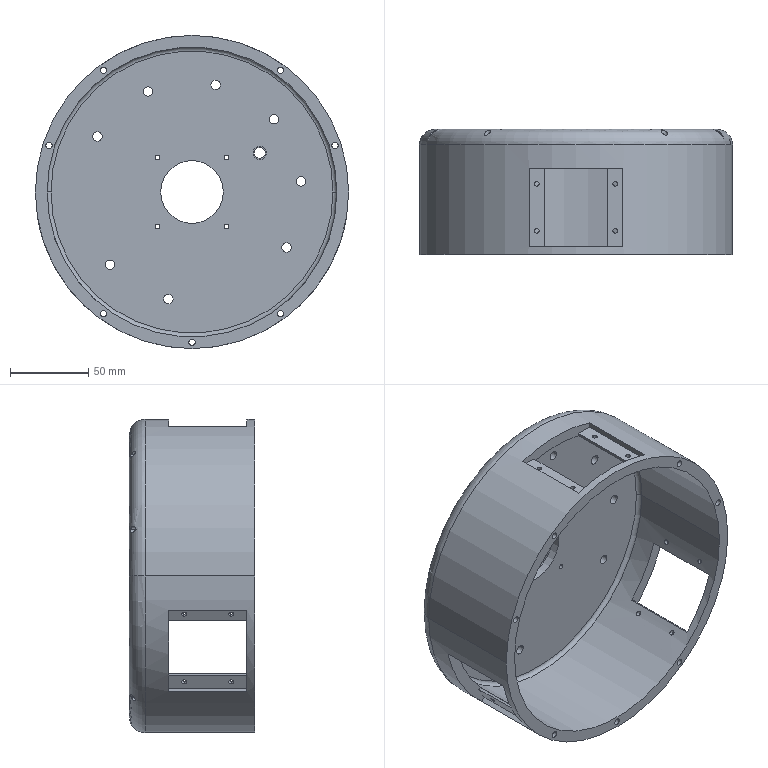Component | SolidWorks | UpperHousing-1 | 1 solid | 106 faces | box 200 x 80 x 200 mm | volume 473499 mm3 | cylinder 72 | plane 28 | torus 6 | commonest cylinder face diameters 3 x32 6 x16 4 x14 8.5 x2 40 x2 185 x2 200 x2 7 x2
build123d program:
from build123d import *

# Parameters (mm, degrees)
SKETCH2_R               = 100
BOSS_EXTRUDE1_DEPTH     = 80
FILLET1_R               = 10
SHELL1_T                = -7.5
CUT_EXTRUDE1_2_REACH    = 164.481
SKETCH3_R               = 2
SKETCH5_W               = 50
SKETCH5_H               = 18.217
CUT_EXTRUDE3_DEPTH      = 20
CIRPATTERN1_COUNT       = 3
SKETCH8_W               = 60
SKETCH8_H               = 50
CUT_EXTRUDE4_DEPTH      = 8
CIRPATTERN2_COUNT       = 3
CUT_EXTRUDE5_REACH      = 232.79
CUT_EXTRUDE5_END_RADIUS = 92.5
SKETCH9_R               = 1.5
CIRPATTERN3_COUNT       = 3
CUT_EXTRUDE6_REACH      = 164.481
SKETCH10_R              = 20
FILLET2_R               = 2
CUT_EXTRUDE7_REACH      = 164.481
SKETCH12_R              = 1.5
CUT_EXTRUDE9_REACH      = 164.481
SKETCH13_R              = 3
CUT_EXTRUDE10_REACH     = 164.481
SKETCH14_R              = 3.5
SKETCH1_R               = 4.25
CUT_EXTRUDE1_DEPTH      = 2.6


with BuildPart() as part:
    # Sketch2 → Boss-Extrude1 (new body)
    with BuildSketch(Plane.XY):
        Circle(SKETCH2_R)
    extrude(amount=BOSS_EXTRUDE1_DEPTH)

    # Fillet1
    fillet1_edges = [part.edges().sort_by_distance(p)[0] for p in [
        (-100, 0, 80),
    ]]
    fillet(fillet1_edges, radius=FILLET1_R)

    # Shell1
    shell1_openings = [part.faces().sort_by_distance(p)[0] for p in [
        (0, 0, 0),
    ]]
    offset(amount=SHELL1_T, openings=shell1_openings, kind=Kind.INTERSECTION)

    # Sketch3 → Cut-Extrude1_2 (cut, up to next)
    with BuildSketch(Plane(origin=(0, 0, 0), x_dir=(-1, 0, 0), z_dir=(0, 0, -1)), mode=Mode.PRIVATE) as cut_extrude1_2_sk1:
        with Locations((0, 96)):
            Circle(SKETCH3_R)
    cut_extrude1_2_tool1 = extrude(cut_extrude1_2_sk1.sketch, amount=-CUT_EXTRUDE1_2_REACH, mode=Mode.PRIVATE) & part.part
    # Sketch3 → Cut-Extrude1_2 (cut, up to next)
    with BuildSketch(Plane(origin=(0, 0, 0), x_dir=(-1, 0, 0), z_dir=(0, 0, -1)), mode=Mode.PRIVATE) as cut_extrude1_2_sk2:
        with Locations((56.427, 77.666)):
            Circle(SKETCH3_R)
    cut_extrude1_2_tool2 = extrude(cut_extrude1_2_sk2.sketch, amount=-CUT_EXTRUDE1_2_REACH, mode=Mode.PRIVATE) & part.part
    # Sketch3 → Cut-Extrude1_2 (cut, up to next)
    with BuildSketch(Plane(origin=(0, 0, 0), x_dir=(-1, 0, 0), z_dir=(0, 0, -1)), mode=Mode.PRIVATE) as cut_extrude1_2_sk3:
        with Locations((91.301, -29.666)):
            Circle(SKETCH3_R)
    cut_extrude1_2_tool3 = extrude(cut_extrude1_2_sk3.sketch, amount=-CUT_EXTRUDE1_2_REACH, mode=Mode.PRIVATE) & part.part
    # Sketch3 → Cut-Extrude1_2 (cut, up to next)
    with BuildSketch(Plane(origin=(0, 0, 0), x_dir=(-1, 0, 0), z_dir=(0, 0, -1)), mode=Mode.PRIVATE) as cut_extrude1_2_sk4:
        with Locations((56.427, -77.666)):
            Circle(SKETCH3_R)
    cut_extrude1_2_tool4 = extrude(cut_extrude1_2_sk4.sketch, amount=-CUT_EXTRUDE1_2_REACH, mode=Mode.PRIVATE) & part.part
    # Sketch3 → Cut-Extrude1_2 (cut, up to next)
    with BuildSketch(Plane(origin=(0, 0, 0), x_dir=(-1, 0, 0), z_dir=(0, 0, -1)), mode=Mode.PRIVATE) as cut_extrude1_2_sk5:
        with Locations((-56.427, -77.666)):
            Circle(SKETCH3_R)
    cut_extrude1_2_tool5 = extrude(cut_extrude1_2_sk5.sketch, amount=-CUT_EXTRUDE1_2_REACH, mode=Mode.PRIVATE) & part.part
    # Sketch3 → Cut-Extrude1_2 (cut, up to next)
    with BuildSketch(Plane(origin=(0, 0, 0), x_dir=(-1, 0, 0), z_dir=(0, 0, -1)), mode=Mode.PRIVATE) as cut_extrude1_2_sk6:
        with Locations((-91.301, -29.666)):
            Circle(SKETCH3_R)
    cut_extrude1_2_tool6 = extrude(cut_extrude1_2_sk6.sketch, amount=-CUT_EXTRUDE1_2_REACH, mode=Mode.PRIVATE) & part.part
    # Sketch3 → Cut-Extrude1_2 (cut, up to next)
    with BuildSketch(Plane(origin=(0, 0, 0), x_dir=(-1, 0, 0), z_dir=(0, 0, -1)), mode=Mode.PRIVATE) as cut_extrude1_2_sk7:
        with Locations((-56.427, 77.666)):
            Circle(SKETCH3_R)
    cut_extrude1_2_tool7 = extrude(cut_extrude1_2_sk7.sketch, amount=-CUT_EXTRUDE1_2_REACH, mode=Mode.PRIVATE) & part.part
    add(cut_extrude1_2_tool1.solids().sort_by_distance((0, 96, 0))[0], mode=Mode.SUBTRACT)
    add(cut_extrude1_2_tool2.solids().sort_by_distance((-56.427, 77.666, 0))[0], mode=Mode.SUBTRACT)
    add(cut_extrude1_2_tool3.solids().sort_by_distance((-91.301, -29.666, 0))[0], mode=Mode.SUBTRACT)
    add(cut_extrude1_2_tool4.solids().sort_by_distance((-56.427, -77.666, 0))[0], mode=Mode.SUBTRACT)
    add(cut_extrude1_2_tool5.solids().sort_by_distance((56.427, -77.666, 0))[0], mode=Mode.SUBTRACT)
    add(cut_extrude1_2_tool6.solids().sort_by_distance((91.301, -29.666, 0))[0], mode=Mode.SUBTRACT)
    add(cut_extrude1_2_tool7.solids().sort_by_distance((56.427, 77.666, 0))[0], mode=Mode.SUBTRACT)

    # Sketch5 → Cut-Extrude3 (cut, symmetric)
    with BuildSketch(Plane(origin=(0, 0, 0), x_dir=(0, 0, -1), z_dir=(1, 0, 0))):
        with Locations((-30, -96.918)):
            Rectangle(SKETCH5_W, SKETCH5_H)
    cut_extrude3 = extrude(amount=CUT_EXTRUDE3_DEPTH, both=True, mode=Mode.SUBTRACT)

    # CirPattern1: Cut-Extrude3 ×3 about axis
    cirpattern1_axis = Axis((0, 0, 0), (0, 0, 1))
    for i in range(1, CIRPATTERN1_COUNT):
        add(cut_extrude3.rotate(cirpattern1_axis, i * 360 / CIRPATTERN1_COUNT), mode=Mode.SUBTRACT)

    # Sketch8 → Cut-Extrude4 (cut)
    with BuildSketch(Plane(origin=(0, -100, 0), x_dir=(1, 0, 0), z_dir=(0, 1, 0))):
        with Locations((0, -30)):
            Rectangle(SKETCH8_W, SKETCH8_H)
    cut_extrude4 = extrude(amount=CUT_EXTRUDE4_DEPTH, mode=Mode.SUBTRACT)

    # CirPattern2: Cut-Extrude4 ×3 about axis
    cirpattern2_axis = Axis((0, 0, 0), (0, 0, 1))
    for i in range(1, CIRPATTERN2_COUNT):
        add(cut_extrude4.rotate(cirpattern2_axis, i * 360 / CIRPATTERN2_COUNT), mode=Mode.SUBTRACT)

    # Cut-Extrude5: up to this cylinder (the profile starts outside it)
    cut_extrude5_end = Plane(origin=(0, 0, 30), z_dir=(0, 0, -1)) * Cylinder(CUT_EXTRUDE5_END_RADIUS, 681.58, mode=Mode.PRIVATE)
    # Sketch9 → Cut-Extrude5 (cut, up to the surface)
    with BuildSketch(Plane.XZ.offset(92), mode=Mode.PRIVATE) as cut_extrude5_sk1:
        with Locations(Location((-25, 45, 0), (0, 0, 270))):
            Circle(SKETCH9_R)
    cut_extrude5_tool1 = extrude(cut_extrude5_sk1.sketch, amount=-CUT_EXTRUDE5_REACH, mode=Mode.PRIVATE) - cut_extrude5_end
    # Sketch9 → Cut-Extrude5 (cut, up to the surface)
    with BuildSketch(Plane.XZ.offset(92), mode=Mode.PRIVATE) as cut_extrude5_sk2:
        with Locations(Location((25, 45, 0), (0, 0, 270))):
            Circle(SKETCH9_R)
    cut_extrude5_tool2 = extrude(cut_extrude5_sk2.sketch, amount=-CUT_EXTRUDE5_REACH, mode=Mode.PRIVATE) - cut_extrude5_end
    # Sketch9 → Cut-Extrude5 (cut, up to the surface)
    with BuildSketch(Plane.XZ.offset(92), mode=Mode.PRIVATE) as cut_extrude5_sk3:
        with Locations(Location((25, 15, 0), (0, 0, 270))):
            Circle(SKETCH9_R)
    cut_extrude5_tool3 = extrude(cut_extrude5_sk3.sketch, amount=-CUT_EXTRUDE5_REACH, mode=Mode.PRIVATE) - cut_extrude5_end
    # Sketch9 → Cut-Extrude5 (cut, up to the surface)
    with BuildSketch(Plane.XZ.offset(92), mode=Mode.PRIVATE) as cut_extrude5_sk4:
        with Locations(Location((-25, 15, 0), (0, 0, 270))):
            Circle(SKETCH9_R)
    cut_extrude5_tool4 = extrude(cut_extrude5_sk4.sketch, amount=-CUT_EXTRUDE5_REACH, mode=Mode.PRIVATE) - cut_extrude5_end
    cut_extrude5 = cut_extrude5_tool1.solids().sort_by_distance((-25, -92, 45))[0] + cut_extrude5_tool2.solids().sort_by_distance((25, -92, 45))[0] + cut_extrude5_tool3.solids().sort_by_distance((25, -92, 15))[0] + cut_extrude5_tool4.solids().sort_by_distance((-25, -92, 15))[0]
    add(cut_extrude5, mode=Mode.SUBTRACT)

    # CirPattern3: Cut-Extrude5 ×3 about axis
    cirpattern3_axis = Axis((0, 0, 80), (0, 0, -1))
    for i in range(1, CIRPATTERN3_COUNT):
        add(cut_extrude5.rotate(cirpattern3_axis, i * 360 / CIRPATTERN3_COUNT), mode=Mode.SUBTRACT)

    # Sketch10 → Cut-Extrude6 (cut, up to next)
    with BuildSketch(Plane.XY.offset(80), mode=Mode.PRIVATE) as cut_extrude6_sk1:
        Circle(SKETCH10_R)
    cut_extrude6_tool1 = extrude(cut_extrude6_sk1.sketch, amount=-CUT_EXTRUDE6_REACH, mode=Mode.PRIVATE) & part.part
    add(cut_extrude6_tool1.solids().sort_by_distance((0, 0, 80))[0], mode=Mode.SUBTRACT)

    # Fillet2
    fillet2_edges = [part.edges().sort_by_distance(p)[0] for p in [
        (-20, 0, 80),
    ]]
    fillet(fillet2_edges, radius=FILLET2_R)

    # Sketch12 → Cut-Extrude7 (cut, up to next)
    with BuildSketch(Plane.XY.offset(80), mode=Mode.PRIVATE) as cut_extrude7_sk1:
        with Locations((-22, 22)):
            Circle(SKETCH12_R)
    cut_extrude7_tool1 = extrude(cut_extrude7_sk1.sketch, amount=-CUT_EXTRUDE7_REACH, mode=Mode.PRIVATE) & part.part
    # Sketch12 → Cut-Extrude7 (cut, up to next)
    with BuildSketch(Plane.XY.offset(80), mode=Mode.PRIVATE) as cut_extrude7_sk2:
        with Locations((22, 22)):
            Circle(SKETCH12_R)
    cut_extrude7_tool2 = extrude(cut_extrude7_sk2.sketch, amount=-CUT_EXTRUDE7_REACH, mode=Mode.PRIVATE) & part.part
    # Sketch12 → Cut-Extrude7 (cut, up to next)
    with BuildSketch(Plane.XY.offset(80), mode=Mode.PRIVATE) as cut_extrude7_sk3:
        with Locations((22, -22)):
            Circle(SKETCH12_R)
    cut_extrude7_tool3 = extrude(cut_extrude7_sk3.sketch, amount=-CUT_EXTRUDE7_REACH, mode=Mode.PRIVATE) & part.part
    # Sketch12 → Cut-Extrude7 (cut, up to next)
    with BuildSketch(Plane.XY.offset(80), mode=Mode.PRIVATE) as cut_extrude7_sk4:
        with Locations((-22, -22)):
            Circle(SKETCH12_R)
    cut_extrude7_tool4 = extrude(cut_extrude7_sk4.sketch, amount=-CUT_EXTRUDE7_REACH, mode=Mode.PRIVATE) & part.part
    add(cut_extrude7_tool1.solids().sort_by_distance((-22, 22, 80))[0], mode=Mode.SUBTRACT)
    add(cut_extrude7_tool2.solids().sort_by_distance((22, 22, 80))[0], mode=Mode.SUBTRACT)
    add(cut_extrude7_tool3.solids().sort_by_distance((22, -22, 80))[0], mode=Mode.SUBTRACT)
    add(cut_extrude7_tool4.solids().sort_by_distance((-22, -22, 80))[0], mode=Mode.SUBTRACT)

    # Sketch13 → Cut-Extrude9 (cut, up to next)
    with BuildSketch(Plane.XY.offset(80), mode=Mode.PRIVATE) as cut_extrude9_sk1:
        with Locations((-28, -64.156)):
            Circle(SKETCH13_R)
    cut_extrude9_tool1 = extrude(cut_extrude9_sk1.sketch, amount=-CUT_EXTRUDE9_REACH, mode=Mode.PRIVATE) & part.part
    # Sketch13 → Cut-Extrude9 (cut, up to next)
    with BuildSketch(Plane.XY.offset(80), mode=Mode.PRIVATE) as cut_extrude9_sk2:
        with Locations((-60.362, -35.445)):
            Circle(SKETCH13_R)
    cut_extrude9_tool2 = extrude(cut_extrude9_sk2.sketch, amount=-CUT_EXTRUDE9_REACH, mode=Mode.PRIVATE) & part.part
    # Sketch13 → Cut-Extrude9 (cut, up to next)
    with BuildSketch(Plane.XY.offset(80), mode=Mode.PRIVATE) as cut_extrude9_sk3:
        with Locations((-52.364, 46.455)):
            Circle(SKETCH13_R)
    cut_extrude9_tool3 = extrude(cut_extrude9_sk3.sketch, amount=-CUT_EXTRUDE9_REACH, mode=Mode.PRIVATE) & part.part
    # Sketch13 → Cut-Extrude9 (cut, up to next)
    with BuildSketch(Plane.XY.offset(80), mode=Mode.PRIVATE) as cut_extrude9_sk4:
        with Locations((-15.058, 68.361)):
            Circle(SKETCH13_R)
    cut_extrude9_tool4 = extrude(cut_extrude9_sk4.sketch, amount=-CUT_EXTRUDE9_REACH, mode=Mode.PRIVATE) & part.part
    # Sketch13 → Cut-Extrude9 (cut, up to next)
    with BuildSketch(Plane.XY.offset(80), mode=Mode.PRIVATE) as cut_extrude9_sk5:
        with Locations((60.362, 35.445)):
            Circle(SKETCH13_R)
    cut_extrude9_tool5 = extrude(cut_extrude9_sk5.sketch, amount=-CUT_EXTRUDE9_REACH, mode=Mode.PRIVATE) & part.part
    # Sketch13 → Cut-Extrude9 (cut, up to next)
    with BuildSketch(Plane.XY.offset(80), mode=Mode.PRIVATE) as cut_extrude9_sk6:
        with Locations((69.669, -6.804)):
            Circle(SKETCH13_R)
    cut_extrude9_tool6 = extrude(cut_extrude9_sk6.sketch, amount=-CUT_EXTRUDE9_REACH, mode=Mode.PRIVATE) & part.part
    # Sketch13 → Cut-Extrude9 (cut, up to next)
    with BuildSketch(Plane.XY.offset(80), mode=Mode.PRIVATE) as cut_extrude9_sk7:
        with Locations((52.364, -46.455)):
            Circle(SKETCH13_R)
    cut_extrude9_tool7 = extrude(cut_extrude9_sk7.sketch, amount=-CUT_EXTRUDE9_REACH, mode=Mode.PRIVATE) & part.part
    # Sketch13 → Cut-Extrude9 (cut, up to next)
    with BuildSketch(Plane.XY.offset(80), mode=Mode.PRIVATE) as cut_extrude9_sk8:
        with Locations((15.058, -68.361)):
            Circle(SKETCH13_R)
    cut_extrude9_tool8 = extrude(cut_extrude9_sk8.sketch, amount=-CUT_EXTRUDE9_REACH, mode=Mode.PRIVATE) & part.part
    add(cut_extrude9_tool1.solids().sort_by_distance((-28, -64.156, 80))[0], mode=Mode.SUBTRACT)
    add(cut_extrude9_tool2.solids().sort_by_distance((-60.362, -35.445, 80))[0], mode=Mode.SUBTRACT)
    add(cut_extrude9_tool3.solids().sort_by_distance((-52.364, 46.455, 80))[0], mode=Mode.SUBTRACT)
    add(cut_extrude9_tool4.solids().sort_by_distance((-15.058, 68.361, 80))[0], mode=Mode.SUBTRACT)
    add(cut_extrude9_tool5.solids().sort_by_distance((60.362, 35.445, 80))[0], mode=Mode.SUBTRACT)
    add(cut_extrude9_tool6.solids().sort_by_distance((69.669, -6.804, 80))[0], mode=Mode.SUBTRACT)
    add(cut_extrude9_tool7.solids().sort_by_distance((52.364, -46.455, 80))[0], mode=Mode.SUBTRACT)
    add(cut_extrude9_tool8.solids().sort_by_distance((15.058, -68.361, 80))[0], mode=Mode.SUBTRACT)

    # Sketch14 → Cut-Extrude10 (cut, up to next)
    with BuildSketch(Plane.XY.offset(80), mode=Mode.PRIVATE) as cut_extrude10_sk1:
        with Locations((43.301, -25)):
            Circle(SKETCH14_R)
    cut_extrude10_tool1 = extrude(cut_extrude10_sk1.sketch, amount=-CUT_EXTRUDE10_REACH, mode=Mode.PRIVATE) & part.part
    add(cut_extrude10_tool1.solids().sort_by_distance((43.301, -25, 80))[0], mode=Mode.SUBTRACT)

    # Sketch1 → Cut-Extrude1 (cut)
    with BuildSketch(Plane(origin=(0, 0, 72.5), x_dir=(-1, 0, 0), z_dir=(0, 0, -1))):
        with Locations((-43.301, -25)):
            Circle(SKETCH1_R)
    extrude(amount=-CUT_EXTRUDE1_DEPTH, mode=Mode.SUBTRACT)


solid = part.part

# Placed as in the assembly
solid = solid.moved(Location((-5.981, 10.507, 160), (-90, 0, 0)))